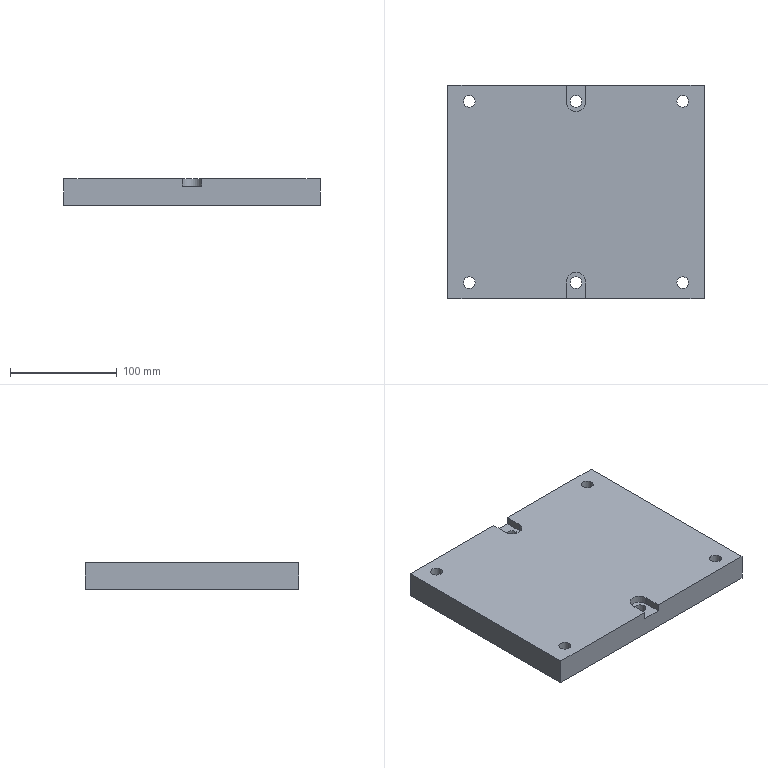Component | NX | BASE_PLATE | 1 solid | 28 faces | volume 1174329 mm3 | plane 16 | cylinder 12 | commonest cylinder face diameters 11 x6 18 x6